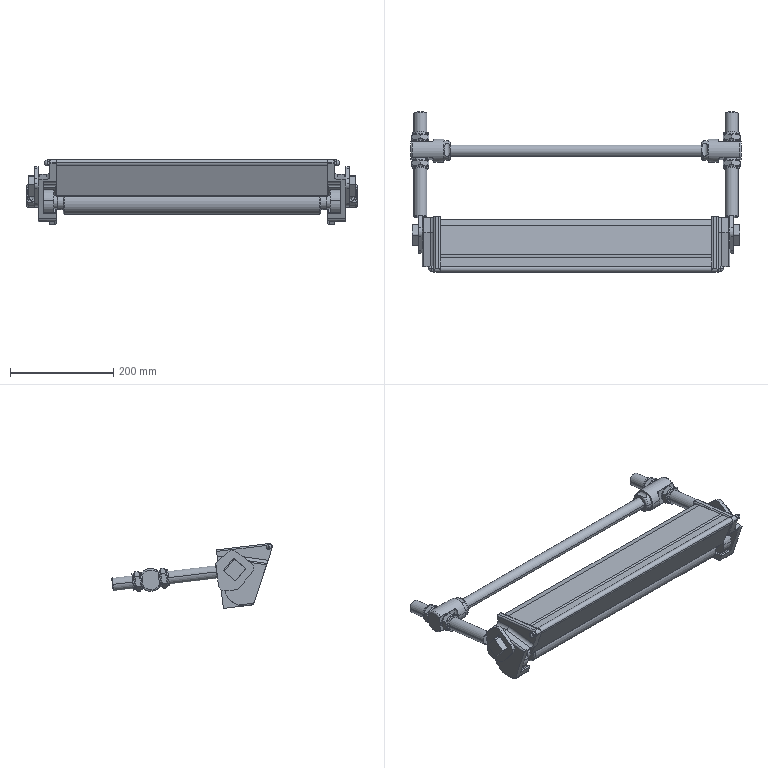Assembly | SolidWorks | mm | 17 component files | 19 solids | 544 faces | box 640.33 x 310.87 x 125.7 mm | volume 2505792 mm3 | plane 178 | cylinder 160 | cone 98 | torus 60 | spline 48 | commonest cylinder face diameters 25.4 x18 12.7 x18 31.75 x16 6.081 x12 26.591 x6 6.528 x6 6.096 x6 49.337 x6
Bill of materials:
LH | 1 |  | Flat plate shaped like an irregular quadrilateral (tapered outline) with a rounded corner that has a small through-hole. A raised flange or ridge runs along the upper edge, and a second slanted rib runs across the face. A rectangular block sticks out from one face, and the opposite side has a curved, partly hollow pocket or boss region.
RH | 1 |  | Tapered quadrilateral plate with a small corner hole. A raised edge flange runs along the top. A cylindrical boss with a through-bore sits on the face, surrounded by a recessed circular or annular groove, and there is a second partial cylindrical boss above it. A rectangular block sticks out from the opposite side, and there is a short cylindrical stub near one end.
DNR-71M20100BBEF2xx-A_500995 | 2 |  | Thin flat plate with a constant thickness. Its outline is an irregular, roughly pentagonal polygon with rounded corners, and a single square or rectangular through-opening sits near the centre.
DNR-71M20100BBEF2xx-A_500996 | 2 |  | Plain solid cylindrical rod of constant diameter with flat ends. The end edges may have a very small chamfer or edge break.
501091 | 1 |  | Long straight extruded profile made of two flat flanges meeting at an angle. At the junction is a rounded boss containing a small round channel that runs the full length, and the inside of the corner has a large fillet. One flange ends in a tapered tip.
DNR-71M20100BBEF2xx-A_500780 | 2 |  | Turned cylindrical body. At one end two parallel flats form a tongue with a round cross-hole through it. Towards the other end there is a stepped shoulder and a reduced-diameter end section with a circumferential groove.
DNR-71M20100BBEF2xx-A_500791 | 4 |  | Short hollow part with a central hexagonal section and a cylindrical collar on both sides. A plain circular through-bore runs along the axis.
502920-TE | 1 |  | Plain solid cylindrical rod or pin with flat ends. Its length is many times its diameter.
509720 | 1 |  | Long slender pin, symmetric end to end. It has a constant-diameter main shank, and each end steps down in diameter twice, ending in a small cylindrical tip.
DNR-71M20100BBEF2xx-A_990608MSS | 2 |  | Hexagonal body with chamfered corners, capped on one side by a rounded dome. There is a small circular feature at the top of the dome.
Mates:
1. distance | DNR-71M20100BBEF2xx-A_500997-1/DNR-71M20100BBEF2xx-A_500996-2 plane at (301.625, 123.459, 137.155) dir (0, 0.1196, 0.9928) | DNR-71M20100BBEF2xx-A_990608MSS-1 plane at (280.672, -179.503, 209.985) dir (0, -0.1196, -0.9928)
2. distance | DNR-71M20100BBEF2xx-A_990608MSS-1 plane at (280.672, -179.503, 209.985) dir (0, -0.9928, 0.1196) | DNR-71M20100BBEF2xx-A_504806-1 plane at (0, 49.445, 146.072) dir (0, -0.9928, 0.1196)
3. concentric | DNR-71M20100BBEF2xx-A_500979-1 face at (262.725, -179.503, 209.985) dir (1, 0, 0) r 3.264 | DNR-71M20100BBEF2xx-A_500979-2 face at (-262.725, -179.503, 209.985) dir (-1, 0, 0) r 3.264
4. angle | DNR-71M20100BBEF2xx-A_500979-1 face at (262.725, -188.831, 217.504) dir (0, 0.1196, 0.9928) | DNR-71M20100BBEF2xx-A_501077-1 face at (-262.725, -152.59, 211.906) dir (0, 0.1369, 0.9906)
5. coincident | DNR-71M20100BBEF2xx-A_500979-2 face at (-262.725, -77.873, 204.136) dir (1, 0, 0) | DNR-71M20100BBEF2xx-A_501077-1 face at (-262.725, -157.474, 146.374) dir (-1, 0, 0)
6. concentric | DNR-71M20100BBEF2xx-A_500979-1 face at (262.725, -179.503, 209.985) dir (1, 0, 0) r 3.264 | DNR-71M20100BBEF2xx-A_501077-1 face at (-302.021, -179.503, 209.985) dir (1, 0, 0) r 3.264
7. coincident | DNR-71M20100BBEF2xx-A_500979-1 face at (275.572, -138.392, 153.864) dir (1, 0, 0) | DNR-71M20100BBEF2xx-A_990608MSS-1 face at (275.572, -179.503, 209.985) dir (-1, 0, 0)
8. concentric | DNR-71M20100BBEF2xx-A_500979-1 face at (262.725, -179.503, 209.985) dir (1, 0, 0) r 3.264 | DNR-71M20100BBEF2xx-A_990608MSS-1 face at (275.572, -179.503, 209.985) dir (1, 0, 0) r 3
9. parallel | DNR-71M20100BBEF2xx-A_500979-1 face at (262.725, -188.831, 217.504) dir (0, 0.1196, 0.9928) | DNR-71M20100BBEF2xx-A_990608MSS-1 plane at (280.672, -179.503, 209.985) dir (0, -0.1196, -0.9928)
10. coincident | DNR-71M20100BBEF2xx-A_500979-2 face at (-275.572, -138.392, 153.864) dir (-1, 0, 0) | DNR-71M20100BBEF2xx-A_990608MSS-2 face at (-275.572, -179.503, 209.985) dir (1, 0, 0)
11. concentric | DNR-71M20100BBEF2xx-A_500979-2 face at (-262.725, -179.503, 209.985) dir (-1, 0, 0) r 3.264 | DNR-71M20100BBEF2xx-A_990608MSS-2 face at (-275.572, -179.503, 209.985) dir (-1, 0, 0) r 3
12. parallel | DNR-71M20100BBEF2xx-A_500979-2 face at (-262.725, -188.831, 217.504) dir (0, 0.1196, 0.9928) | DNR-71M20100BBEF2xx-A_990608MSS-2 plane at (-280.672, -179.503, 209.985) dir (0, -0.1196, -0.9928)
13. distance | DNR-71M20100BBEF2xx-A_500997-1/DNR-71M20100BBEF2xx-A_500996-2 face at (301.625, 123.459, 137.155) dir (0, 0.9928, -0.1196) | DNR-71M20100BBEF2xx-A_504806-1/DNR-71M20100BBEF2xx-A_500780-1 face at (275.717, 67.067, 159.616) dir (0, 0.9928, -0.1196)
14. concentric | DNR-71M20100BBEF2xx-A_500997-2/DNR-71M20100BBEF2xx-A_500996-2 face at (-301.625, 123.459, 137.155) dir (0, 0.9928, -0.1196) r 12.7 | DNR-71M20100BBEF2xx-A_504806-1/DNR-71M20100BBEF2xx-A_500791-2 face at (-301.625, 33.684, 147.971) dir (0, -0.9928, 0.1196) r 12.7
15. coincident | DNR-71M20100BBEF2xx-A_500997-1/DNR-71M20100BBEF2xx-A_500996-2 face at (301.625, 123.459, 137.155) dir (0, 0.9928, -0.1196) | DNR-71M20100BBEF2xx-A_500997-2/DNR-71M20100BBEF2xx-A_500996-2 face at (-301.625, 123.459, 137.155) dir (0, 0.9928, -0.1196)
16. coincident | DNR-71M20100BBEF2xx-A_500997-1 plane at (301.625, -113.427, 165.976) dir (0, 0.1196, 0.9928) | DNR-71M20100BBEF2xx-A_500997-2 plane at (-301.625, -113.427, 165.976) dir (0, 0.1196, 0.9928)
17. coincident | DNR-71M20100BBEF2xx-A_500979-1 face at (262.725, -188.831, 217.504) dir (0, 0.1196, 0.9928) | DNR-71M20100BBEF2xx-A_500979-2 face at (-262.725, -188.831, 217.504) dir (0, 0.1196, 0.9928)
18. concentric | DNR-71M20100BBEF2xx-A_500979-2 face at (-268.122, -131.119, 133.8) dir (-1, 0, 0) r 24.668 | DNR-71M20100BBEF2xx-A_509706-1 face at (276.225, -131.119, 133.8) dir (1, 0, 0) r 23.812
19. coincident | DNR-71M20100BBEF2xx-A_504806-1 plane at (0, 49.445, 146.072) dir (1, 0, 0) | DNR-71M20100BBEF2xx-A_509706-1 plane at (0, -131.119, 133.8) dir (1, 0, 0)
20. parallel | DNR-71M20100BBEF2xx-A_509706-1 plane at (0, -131.119, 133.8) dir (0, 1, 0) | assembly plane at (0, 0, 0) dir (0, 1, 0)
21. concentric | DNR-71M20100BBEF2xx-A_500997-1/DNR-71M20100BBEF2xx-A_500996-2 face at (301.625, 123.459, 137.155) dir (0, 0.9928, -0.1196) r 12.7 | DNR-71M20100BBEF2xx-A_504806-1/DNR-71M20100BBEF2xx-A_500791-4 face at (301.625, 33.684, 147.971) dir (0, -0.9928, 0.1196) r 12.7
22. concentric | DNR-71M20100BBEF2xx-A_500997-2/DNR-71M20100BBEF2xx-A_500996-2 face at (-301.625, 123.459, 137.155) dir (0, 0.9928, -0.1196) r 12.7 | DNR-71M20100BBEF2xx-A_504806-1/DNR-71M20100BBEF2xx-A_500791-2 face at (-301.625, 33.684, 147.971) dir (0, -0.9928, 0.1196) r 12.7
23. coincident | DNR-71M20100BBEF2xx-A_500997-2/DNR-71M20100BBEF2xx-A_500995-1 face at (-298.45, -109.257, 189.258) dir (1, 0, 0) | DNR-71M20100BBEF2xx-A_500979-2 face at (-298.45, -77.873, 204.136) dir (-1, 0, 0)
24. coincident | DNR-71M20100BBEF2xx-A_500997-1/DNR-71M20100BBEF2xx-A_500995-1 face at (298.45, -109.257, 189.258) dir (-1, 0, 0) | DNR-71M20100BBEF2xx-A_500979-1 face at (298.45, -77.873, 204.136) dir (1, 0, 0)
25. coincident | DNR-71M20100BBEF2xx-A_500995-1 face at (-34.925, -39.116, -3.175) dir (-1, 0, 0) | DNR-71M20100BBEF2xx-A_500996-2 face at (-34.925, -0.2794, 0) dir (1, 0, 0)
26. coincident | DNR-71M20100BBEF2xx-A_500995-1 plane at (0, 0, 0) dir (0, 0, 1) | DNR-71M20100BBEF2xx-A_500996-2 plane at (-238.633, -0.2794, 0) dir (0, 0, 1)
27. distance | DNR-71M20100BBEF2xx-A_500995-1 face at (-3.399, -39.116, -3.175) dir (0, -1, 0) | DNR-71M20100BBEF2xx-A_500996-2 plane at (-238.633, -0.2794, 0) dir (0, 1, 0)
28. concentric | DNR-71M20100BBEF2xx-A_502906-1 face at (0, 0, 263.525) dir (0, 0, -1) r 11.113 | DNR-71M20100BBEF2xx-A_500780-1 face at (0, 0, 320.167) dir (0, 0, -1) r 22.225
29. parallel | DNR-71M20100BBEF2xx-A_500780-1 plane at (0, 0, 243.967) dir (1, 0, 0) | DNR-71M20100BBEF2xx-A_504806 plane at (0, 0, 0) dir (1, 0, 0)
30. concentric | DNR-71M20100BBEF2xx-A_502906-1 face at (0, 0, 263.525) dir (0, 0, -1) r 11.113 | DNR-71M20100BBEF2xx-A_500780-2 face at (0, 0, -320.167) dir (0, 0, 1) r 22.225
31. parallel | DNR-71M20100BBEF2xx-A_500780-1 face at (15.875, -15.554, 275.717) dir (1, 0, 0) | DNR-71M20100BBEF2xx-A_500780-2 face at (15.875, -15.554, -275.717) dir (1, 0, 0)
32. distance | DNR-71M20100BBEF2xx-A_500780-1 plane at (0, 0, 301.625) dir (0, 0, 1) | DNR-71M20100BBEF2xx-A_504806 plane at (0, 0, 0) dir (0, 0, 1)
33. distance | DNR-71M20100BBEF2xx-A_500780-2 plane at (0, 0, -301.625) dir (0, 0, -1) | DNR-71M20100BBEF2xx-A_504806 plane at (0, 0, 0) dir (0, 0, 1)
34. coincident | DNR-71M20100BBEF2xx-A_500780-2 face at (-15.875, -15.554, -275.717) dir (-1, 0, 0) | DNR-71M20100BBEF2xx-A_500791-1 face at (-15.875, 0, -301.625) dir (1, 0, 0)
35. coincident | DNR-71M20100BBEF2xx-A_500780-2 plane at (0, 0, -301.625) dir (0, 0, -1) | DNR-71M20100BBEF2xx-A_500791-1 plane at (-25.4, 0, -301.625) dir (0, 0, -1)
36. coincident | DNR-71M20100BBEF2xx-A_500780-2 plane at (0, 0, -243.967) dir (0, -1, 0) | DNR-71M20100BBEF2xx-A_500791-1 plane at (-25.4, 0, -301.625) dir (0, -1, 0)